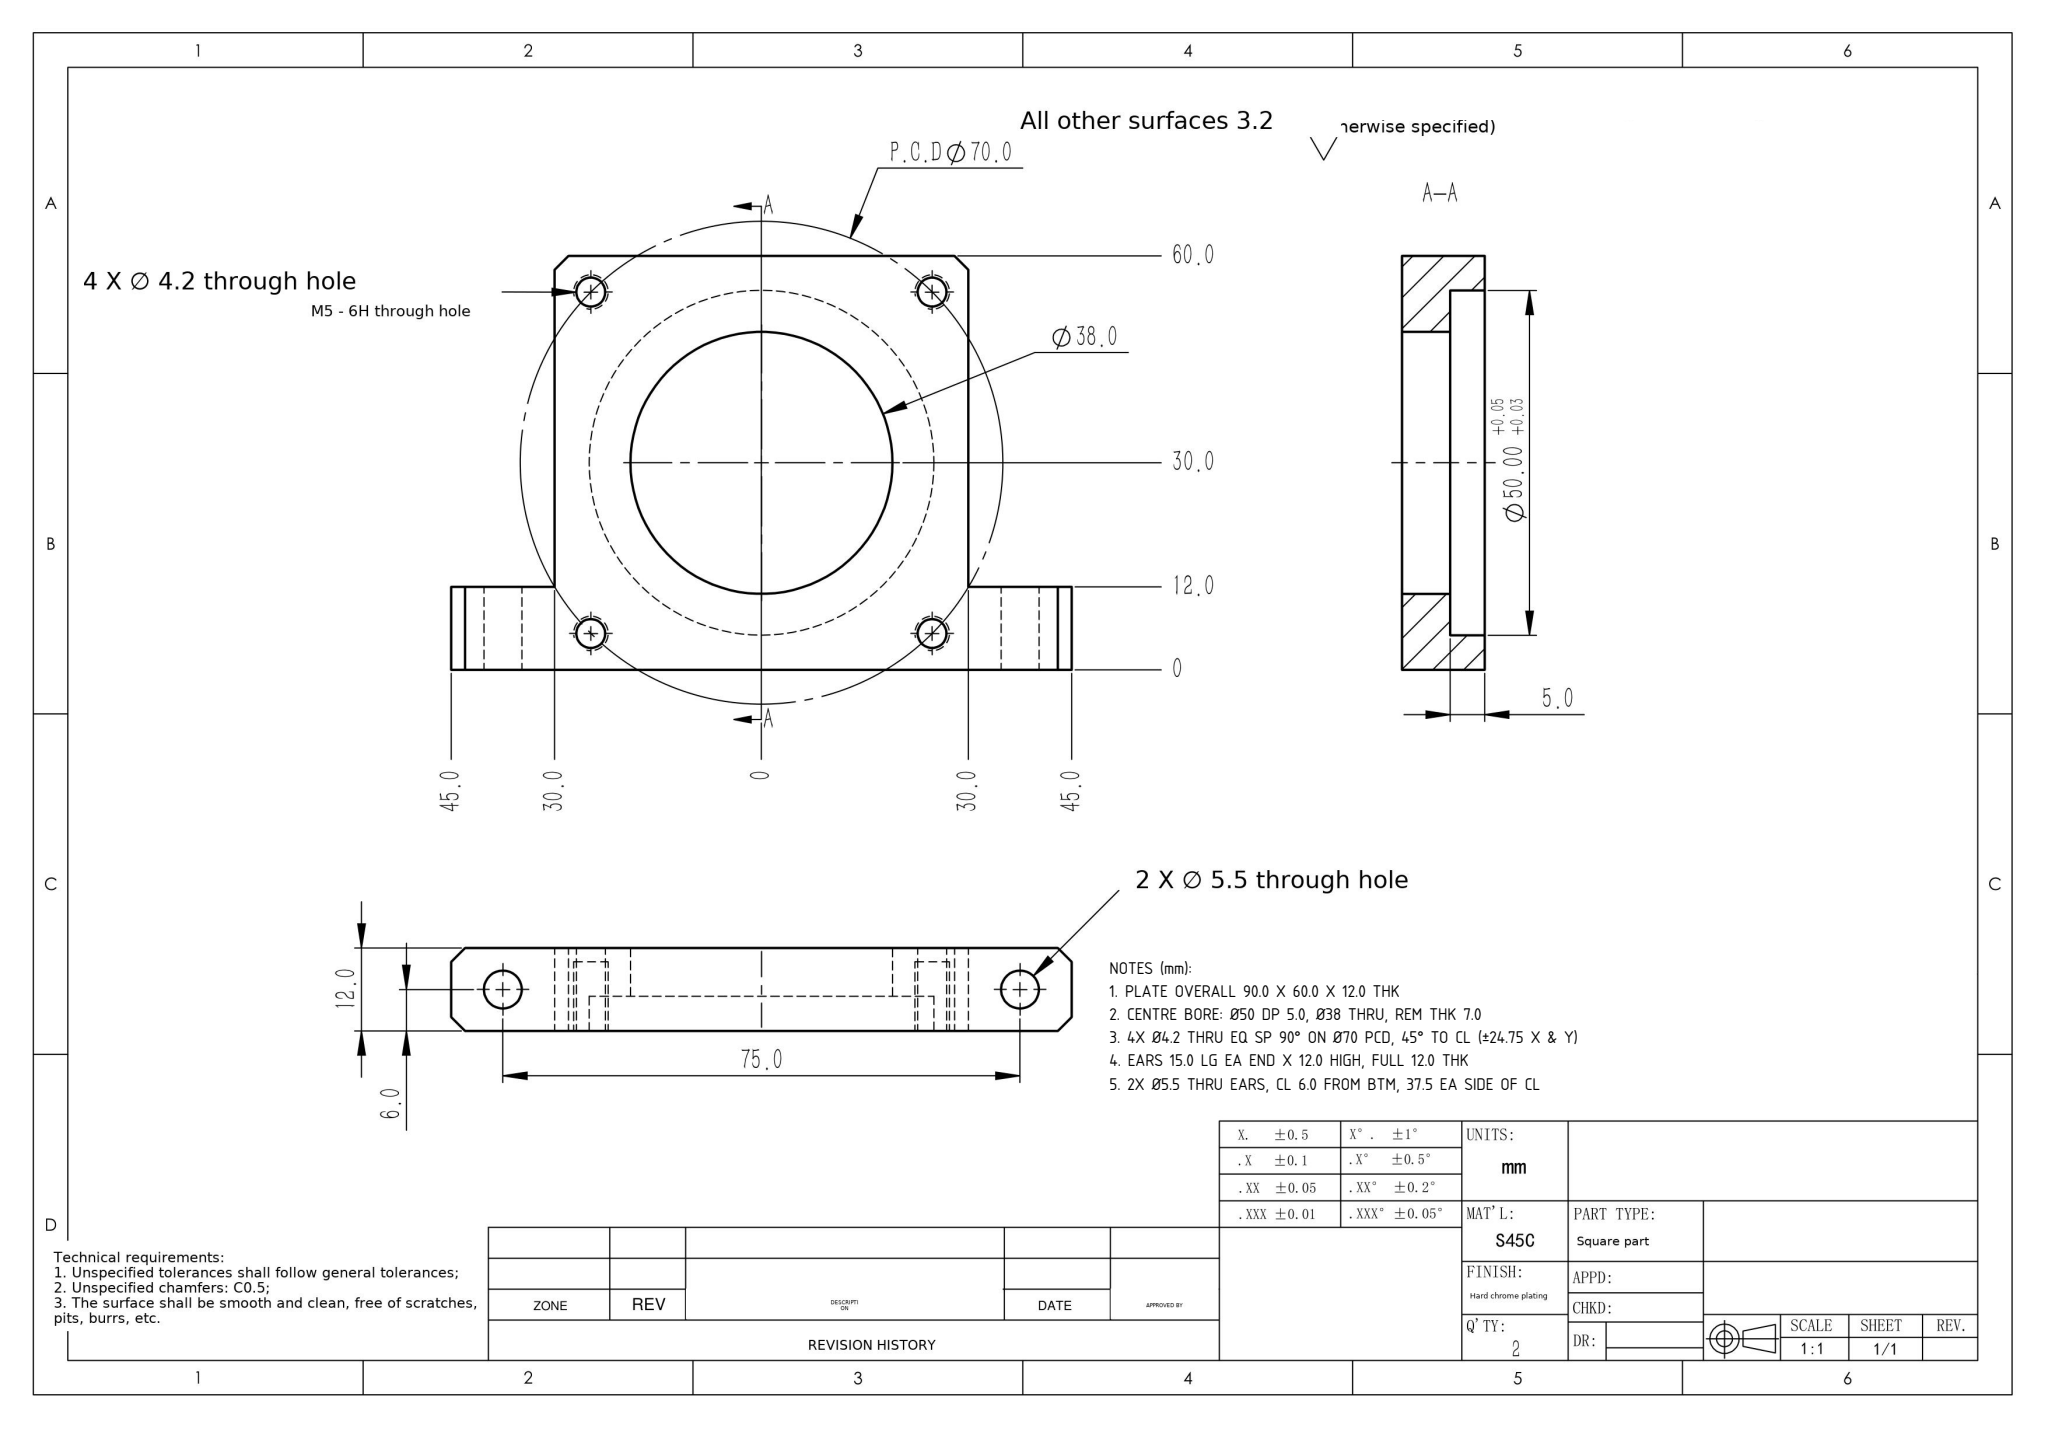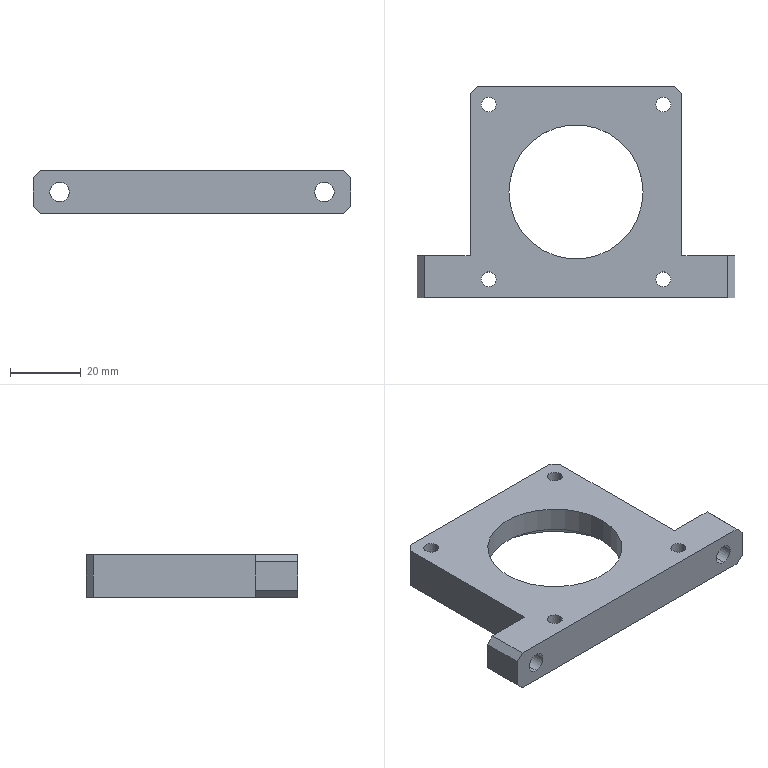Part | SolidWorks | mm | 1 solid | 33 faces | box 90 x 60 x 12 mm | volume 28385 mm3 | plane 17 | cylinder 16 | commonest cylinder face diameters 4.2 x8 5.5 x4 38 x2 50 x2
Drawing notes:
PLATE OVERALL 90.0 X 60.0 X 12.0 THK | from the solid: bbox_xyz 90.0 x 60.0 x 12.0
CENTRE BORE: Ø50 DP 5.0, Ø38 THRU, REM THK 7.0 | from the solid: Ø50 len 5.0 & Ø38 len 7.0 coaxial at (45,30); z-planes 0/5/12
4X Ø4.2 THRU EQ SP 90° ON Ø70 PCD, 45° TO CL (±24.75 X & Y) | from the solid: Ø4.2 z-holes at (20.25,5.25),(20.25,54.75),(69.75,5.25),(69.75,54.75); ctr 45,30
EARS 15.0 LG EA END X 12.0 HIGH, FULL 12.0 THK | from the solid: x-planes 0/15/75/90, y-planes 0/12, bbox z=12.0
2X Ø5.5 THRU EARS, CL 6.0 FROM BTM, 37.5 EA SIDE OF CL | from the solid: Ø5.5 y-axis holes at x=7.5 & 82.5, z=6.0, len 12.0; part CL x=45
build123d program:
from build123d import *

# Parameters (mm, degrees)
SKETCH1_W            = 90
SKETCH1_H            = 60
BOSS_EXTRUDE1_DEPTH  = 12
SKETCH2_W            = 15
SKETCH2_H            = 48
CUT_EXTRUDE1_DEPTH   = 56.399
SKETCH3_R            = 25
CUT_EXTRUDE2_DEPTH   = 5
SKETCH8_R            = 19
CUT_EXTRUDE3_DEPTH   = 56.399
M5_CLEARANCE_HOLE1_D = 5.5
M5_TAPPED_HOLE1_D    = 4.2
CHAMFER1_SIZE        = 2


with BuildPart() as part:
    # Sketch1 → Boss-Extrude1 (new body)
    with BuildSketch(Plane.XY):
        Rectangle(SKETCH1_W, SKETCH1_H)
    extrude(amount=BOSS_EXTRUDE1_DEPTH)

    # Sketch2 → Cut-Extrude1 (cut, through all)
    with BuildSketch(Plane.XY.offset(12)):
        with Locations((-37.5, 6)):
            Rectangle(SKETCH2_W, SKETCH2_H)
        with Locations((37.5, 6)):
            Rectangle(SKETCH2_W, SKETCH2_H)
    extrude(amount=-CUT_EXTRUDE1_DEPTH, mode=Mode.SUBTRACT)

    # Sketch3 → Cut-Extrude2 (cut)
    with BuildSketch(Plane.XY):
        Circle(SKETCH3_R)
    extrude(amount=CUT_EXTRUDE2_DEPTH, mode=Mode.SUBTRACT)

    # Sketch8 → Cut-Extrude3 (cut, through all)
    with BuildSketch(Plane(origin=(0, 0, 0), x_dir=(-1, 0, 0), z_dir=(0, 0, -1))):
        Circle(SKETCH8_R)
    extrude(amount=-CUT_EXTRUDE3_DEPTH, mode=Mode.SUBTRACT)

    # M5 Clearance Hole1 (through all)
    with Locations(Plane(origin=(0, -18, 0), x_dir=(1, 0, 0), z_dir=(0, 1, 0))):
        with Locations((-37.5, -6), (37.5, -6)):
            Hole(M5_CLEARANCE_HOLE1_D / 2)

    # M5 Tapped Hole1 (through all)
    with Locations(Plane(origin=(0, 0, 0), x_dir=(-1, 0, 0), z_dir=(0, 0, -1))):
        with Locations((-24.749, 24.749), (24.749, 24.749), (24.749, -24.749), (-24.749, -24.749)):
            Hole(M5_TAPPED_HOLE1_D / 2)

    # Chamfer1
    chamfer1_edges = [part.edges().sort_by_distance(p)[0] for p in [
        (-45, -24, 0),
        (-45, -24, 12),
        (-30, 30, 6),
        (30, 30, 6),
        (45, -24, 12),
        (45, -24, 0),
    ]]
    chamfer(chamfer1_edges, length=CHAMFER1_SIZE)


solid = part.part